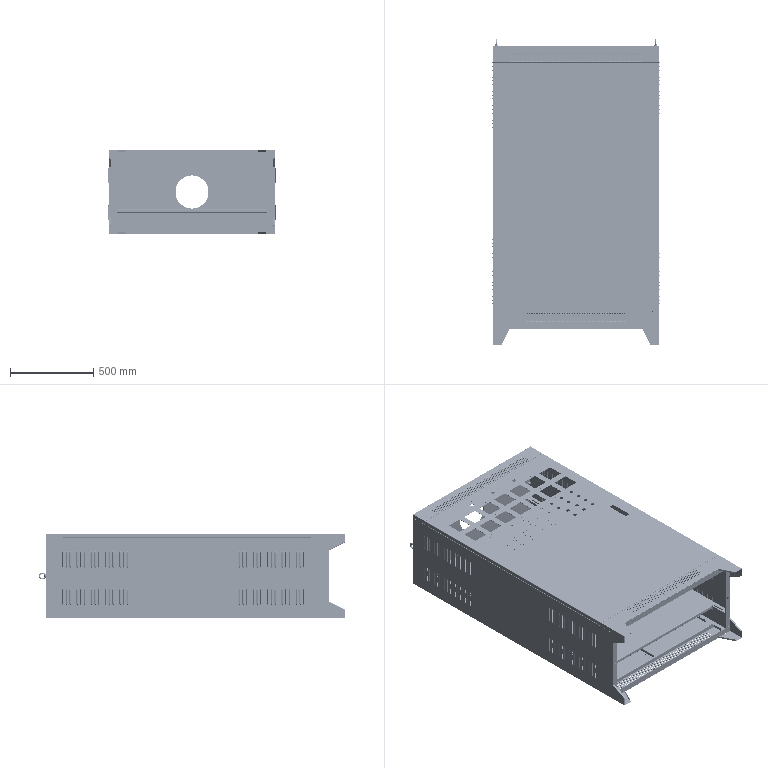Assembly | SolidWorks | mm | 36 component files | 42 solids | 7368 faces | box 1010 x 1843.66 x 510 mm | volume 13388712 mm3 | cylinder 3454 | plane 2960 | torus 460 | sphere 436 | spline 48 | cone 10 | commonest cylinder face diameters 6 x1184 8.4 x592 3.6 x592 3.4 x224 10 x216 8 x118 7.6 x108 12.4 x108
Bill of materials:
27x100IronPlate | 4 |  | Thin flat rectangular plate or strip, elongated, with no visible holes or cutouts.
AirFurnaceElectricalCabinet-AngleIronFrame | 2 |  | Rectangular open frame made of four straight bars of square-ish section, with one small round through-hole in each short side member.
AirFurnaceElectricalCabinet-DoorPanel | 1 |  | Flat rectangular plate with a cutout pattern in one region: two rows of seven square openings, a grid of small round holes below them, three larger round holes above, many tiny holes around the square openings, and one narrow rectangular slot.
AirFurnaceElectricalCabinet-WireDuct | 3 |  | Long, slender, shallow U-section (channel) profile of constant cross-section, with rounded inside corners.
AirFurnaceElectricalCabinet-WiringBoard | 2 |  | Thin sheet bent into a U shape: a flat base with two upright end flanges and small inside bend radii.
DoorPanelReinforcementPlate-L590 | 1 |  | Long hat-section (top-hat) rail: a recessed central channel with outward horizontal flanges on both sides and rounded bends.
DoorPanelReinforcementPlate-L790 | 1 |  | Long hat-section rail with a deep central channel, outward flanges and rounded bends; similar to the previous hat profile but longer relative to its section.
AirFurnaceElectricalCabinet-ElectricalPanel | 1 |  | Large flat rectangular sheet panel with shallow turned-down edges or lips, and small slots or notches spaced along the two long edges.
ElectricalPanelReinforcementPlate-L1425 | 2 |  | Long, narrow hat-section rail with outward flanges and rounded bends; a slimmer, longer version of the hat profile.
AirFurnaceElectricalCabinet-FrontDoorLowerPlate | 1 |  | Long, formed sheet strip with a stepped (Z-like) cross-section and a long row of narrow, closely spaced slots (louvre or vent pattern) in a slightly offset or embossed region.
AirFurnaceElectricalCabinet-LeftSidePlate | 1 |  | Rectangular sheet panel with short return flanges along the top and bottom long edges, and four groups of vertical louvre slots (two upper and two lower rows near each end), each group made of repeated sets of three slots.
AirFurnaceElectricalCabinet-RearLowerPlate | 1 |  | Long formed sheet strip with a flat base, a raised embossed area containing a long row of narrow transverse slots, and an upright side wall with a top flange turned outward at one edge.
AirFurnaceElectricalCabinet-RearSealingPlate | 1 |  | Thin flat rectangular plate with a small through hole near each of the four corners and a narrow stepped or lipped border around the edge.
DoorPanelReinforcementPlate-L1490 | 1 |  | Long, straight, constant-section profile with a hat (omega) cross-section: a raised flat top, two vertical walls, and a flat outward flange on each side, with rounded bends.
AirFurnaceElectricalCabinet-RightSidePlate | 1 |  | Long, sheet-metal-style panel with a C-like section. A flat web has short return flanges along the top and bottom edges, one with an extra small lip. Each end region has louver groups: two rows of four sets, each set made of three narrow vertical slots.
AirFurnaceElectricalCabinet-TopPlate | 1 |  | Channel-shaped sheet-metal bracket. A tall flat web has one large central round hole and a small round hole near each end. The top and bottom flanges have stepped returns, and each flange has a long row of small perforations.
BaseFoot-H100 | 4 |  | Bent sheet-metal piece with a tapered outline: a wide flange on top, a vertical web, and a short bottom flange. One edge is cut at an angle, so the plan outline is a trapezoid.
LargeLiftingRing | 2 |  | Eye-bolt-shaped part: a straight shank with external threads, a collar with a flared base, and a circular ring eye in a plane that contains the shank axis.
SealingPlateAngleIron | 4 |  | Flat right-triangle plate of uniform thickness with one round through hole near the corner where the two straight edges meet at a right angle.
UniversalAngleIron38x38x1690 | 2 |  | Long straight angle (L-section) with legs of about equal length, and a row of evenly spaced elongated slots along one leg.
Mates:
1. distance | AirFurnaceElectricalCabinet-LeftSidePlate-1 face at (-500, 1700, 229.2) dir (-1, 0, 0) | assembly plane at (0, 0, 0) dir (1, 0, 0)
2. coincident | AirFurnaceElectricalCabinet-AngleIronFrame-1 face at (-498.8, 0, 253.5) dir (0, -1, 0) | AirFurnaceElectricalCabinet-LeftSidePlate-1 face at (-498.05, 0, -253.6) dir (0, -1, 0)
3. distance | assembly plane at (0, 0, 0) dir (1, 0, 0) | AirFurnaceElectricalCabinet-RightSidePlate-1 face at (500, 1700, 229.2) dir (1, 0, 0)
4. coincident | AirFurnaceElectricalCabinet-AngleIronFrame-1 face at (495.5, 0, 253.5) dir (0, -1, 0) | AirFurnaceElectricalCabinet-RightSidePlate-1 face at (498.05, 0, 228) dir (0, -1, 0)
5. coincident | AirFurnaceElectricalCabinet-FrontDoorLowerPlate-1 plane at (0, 0, 255) dir (1, 0, 0) | assembly plane at (0, 0, 0) dir (1, 0, 0)
6. coincident | AirFurnaceElectricalCabinet-AngleIronFrame-1 face at (498.8, 0, 253.5) dir (0, -1, 0) | AirFurnaceElectricalCabinet-FrontDoorLowerPlate-1 plane at (0, 0, 255) dir (0, 1, 0)
7. distance | AirFurnaceElectricalCabinet-FrontDoorLowerPlate-1 face at (498.8, 0, 255) dir (0, 0, 1) | assembly plane at (0, 0, 0) dir (0, 0, 1)
8. coincident | AirFurnaceElectricalCabinet-RightSidePlate-1 face at (460, 1700, 229.2) dir (0, 0, 1) | AirFurnaceElectricalCabinet-FrontDoorLowerPlate-1 face at (498.8, 100, 229.2) dir (0, 0, 1)
9. coincident | AirFurnaceElectricalCabinet-LeftSidePlate-1 face at (-460, 1700, 229.2) dir (0, 0, 1) | AirFurnaceElectricalCabinet-FrontDoorLowerPlate-1 face at (498.8, 100, 229.2) dir (0, 0, 1)
10. coincident | AirFurnaceElectricalCabinet-TopPlate-2 plane at (0, 1700, 0) dir (1, 0, 0) | assembly plane at (0, 0, 0) dir (1, 0, 0)
11. coincident | AirFurnaceElectricalCabinet-FrontDoorLowerPlate-1 face at (498.8, 0, 255) dir (0, 0, 1) | AirFurnaceElectricalCabinet-TopPlate-2 face at (498.8, 1600, 255) dir (0, 0, 1)
12. distance | AirFurnaceElectricalCabinet-AngleIronFrame-1 face at (498.8, 0, 253.5) dir (0, -1, 0) | AirFurnaceElectricalCabinet-TopPlate-2 face at (498.8, 1700, 255) dir (0, 1, 0)
13. coincident | AirFurnaceElectricalCabinet-RearLowerPlate-1 plane at (0, 0, -255) dir (1, 0, 0) | assembly plane at (0, 0, 0) dir (1, 0, 0)
14. coincident | AirFurnaceElectricalCabinet-AngleIronFrame-1 face at (495.5, 0, -253.5) dir (0, -1, 0) | AirFurnaceElectricalCabinet-RearLowerPlate-1 plane at (0, 0, -255) dir (0, 1, 0)
15. coincident | AirFurnaceElectricalCabinet-TopPlate-2 face at (498.8, 1700, -255) dir (0, 0, -1) | AirFurnaceElectricalCabinet-RearLowerPlate-1 face at (460, 0, -255) dir (0, 0, -1)
16. coincident | AirFurnaceElectricalCabinet-TopPlate-2 face at (498.8, 1698.8, 255) dir (0, -1, 0) | AirFurnaceElectricalCabinet-AngleIronFrame-2 face at (-495.5, 1698.8, -253.8) dir (0, 1, 0)
17. coincident | AirFurnaceElectricalCabinet-AngleIronFrame-2 plane at (0, 1698.8, -0.3) dir (-1, 0, 0) | assembly plane at (0, 0, 0) dir (1, 0, 0)
18. coincident | AirFurnaceElectricalCabinet-TopPlate-2 face at (498.8, 1700, -253.8) dir (0, 0, 1) | AirFurnaceElectricalCabinet-AngleIronFrame-2 face at (-495.5, 1660.8, -253.8) dir (0, 0, -1)
19. coincident | AirFurnaceElectricalCabinet-AngleIronFrame-1 face at (498.8, 3, 253.5) dir (0, 1, 0) | UniversalAngleIron38x38x1690-1 face at (457.8, 3, -108) dir (0, -1, 0)
20. distance | UniversalAngleIron38x38x1690-1 face at (495.8, 1693, -105) dir (0, 0, 1) | AirFurnaceElectricalCabinet-TopPlate-2 face at (498.8, 1700, -255) dir (0, 0, -1)
21. coincident | AirFurnaceElectricalCabinet-ElectricalPanelAssembly-1 plane at (0, 835.8, -103.5) dir (1, 0, 0) | assembly plane at (0, 0, 0) dir (1, 0, 0)
22. coincident | UniversalAngleIron38x38x1690-2 face at (-495.8, 3, -105) dir (0, 0, 1) | AirFurnaceElectricalCabinet-ElectricalPanelAssembly-1/AirFurnaceElectricalCabinet-ElectricalPanel-1 face at (487.5, 1560.8, -105) dir (0, 0, -1)
23. coincident | AirFurnaceElectricalCabinet-RearLowerPlate-1 face at (460, 110.8, -228) dir (0, 1, 0) | AirFurnaceElectricalCabinet-ElectricalPanelAssembly-1/AirFurnaceElectricalCabinet-ElectricalPanel-1 face at (487.5, 110.8, -103.5) dir (0, -1, 0)
24. coincident | AirFurnaceElectricalCabinet-FrontDoorLowerPlate-1 face at (498.8, 0, 255) dir (0, 0, 1) | BaseFoot-H100-1 face at (-500, -100, 255) dir (0, 0, 1)
25. coincident | AirFurnaceElectricalCabinet-LeftSidePlate-1 face at (-500, 1700, 229.2) dir (-1, 0, 0) | BaseFoot-H100-1 face at (-500, -100, 155) dir (-1, 0, 0)
26. coincident | AirFurnaceElectricalCabinet-RightSidePlate-1 face at (500, 1700, 229.2) dir (1, 0, 0) | BaseFoot-H100-2 face at (500, -100, 255) dir (1, 0, 0)
27. coincident | AirFurnaceElectricalCabinet-FrontDoorLowerPlate-1 face at (498.8, 0, 255) dir (0, 0, 1) | BaseFoot-H100-2 face at (400, -100, 255) dir (0, 0, 1)
28. coincident | AirFurnaceElectricalCabinet-AngleIronFrame-1 face at (498.8, 0, 253.5) dir (0, -1, 0) | BaseFoot-H100-2 edge at (498.8, 0, 252.8) dir (0, 0, -1)
29. coincident | AirFurnaceElectricalCabinet-AngleIronFrame-1 face at (495.5, 0, 253.5) dir (0, -1, 0) | BaseFoot-H100-1 face at (-497.8, 0, 252.8) dir (0, 1, 0)
30. coincident | AirFurnaceElectricalCabinet-RightSidePlate-1 face at (500, 1700, 229.2) dir (1, 0, 0) | BaseFoot-H100-3 face at (500, -100, -155) dir (1, 0, 0)
31. coincident | AirFurnaceElectricalCabinet-RearLowerPlate-1 face at (460, 0, -255) dir (0, 0, -1) | BaseFoot-H100-3 face at (500, -100, -255) dir (0, 0, -1)
32. coincident | AirFurnaceElectricalCabinet-AngleIronFrame-1 face at (495.5, 0, -253.5) dir (0, -1, 0) | BaseFoot-H100-3 face at (497.8, 0, -252.8) dir (0, 1, 0)
33. coincident | AirFurnaceElectricalCabinet-LeftSidePlate-1 face at (-500, 1700, 229.2) dir (-1, 0, 0) | BaseFoot-H100-4 face at (-500, -100, -255) dir (-1, 0, 0)
34. coincident | AirFurnaceElectricalCabinet-RearLowerPlate-1 face at (460, 0, -255) dir (0, 0, -1) | BaseFoot-H100-4 face at (-400, -100, -255) dir (0, 0, -1)
35. coincident | AirFurnaceElectricalCabinet-AngleIronFrame-1 face at (495.5, 0, -253.5) dir (0, -1, 0) | BaseFoot-H100-4 edge at (-400, 0, -255) dir (-1, 0, 0)
36. coincident | AirFurnaceElectricalCabinet-TopPlate-2 face at (498.8, 1600, 255) dir (0, 0, 1) | AirFurnaceElectricalCabinet-DoorPanelAssembly-1/AirFurnaceElectricalCabinet-DoorPanel-1 face at (0, 850, 255) dir (0, 0, 1)
37. distance | AirFurnaceElectricalCabinet-FrontDoorLowerPlate-1 face at (498.8, 100, 255) dir (0, 1, 0) | AirFurnaceElectricalCabinet-DoorPanelAssembly-1/AirFurnaceElectricalCabinet-DoorPanel-1 face at (0, 102, 255) dir (0, -1, 0)
38. concentric | AirFurnaceElectricalCabinet-FrontDoorLowerPlate-1 face at (-493, 98.8, 248) dir (0, 1, 0) r 3.25 | AirFurnaceElectricalCabinet-DoorPanelAssembly-1/AirFurnaceElectricalCabinet-DoorPanel-1 face at (-493, 101.996, 248) dir (0, 1, 0) r 3.25
39. coincident | AirFurnaceElectricalCabinet-LeftSidePlate-1 face at (-460, 1700, -227.8) dir (0, 0, 1) | SealingPlateAngleIron-1 face at (-460, 100, -227.8) dir (0, 0, -1)
40. coincident | AirFurnaceElectricalCabinet-LeftSidePlate-1 face at (-460, 1700, -254.8) dir (1, 0, 0) | SealingPlateAngleIron-1 face at (-460, 165, -227.8) dir (-1, 0, 0)
41. coincident | AirFurnaceElectricalCabinet-RearLowerPlate-1 face at (460, 100, -255) dir (0, 1, 0) | SealingPlateAngleIron-1 face at (-460, 100, -227.8) dir (0, -1, 0)
42. coincident | SealingPlateAngleIron-1 face at (-460, 100, -227.8) dir (0, 0, -1) | SealingPlateAngleIron-2 face at (-460, 1600, -227.8) dir (0, 0, -1)
43. coincident | AirFurnaceElectricalCabinet-TopPlate-2 face at (498.8, 1600, -255) dir (0, -1, 0) | SealingPlateAngleIron-2 face at (-395, 1600, -227.8) dir (0, 1, 0)
44. coincident | AirFurnaceElectricalCabinet-LeftSidePlate-1 face at (-460, 1700, -254.8) dir (1, 0, 0) | SealingPlateAngleIron-2 face at (-460, 1600, -227.8) dir (-1, 0, 0)
45. coincident | AirFurnaceElectricalCabinet-RearSealingPlateAssembly-1 plane at (0, 850, -255) dir (-1, 0, 0) | assembly plane at (0, 0, 0) dir (1, 0, 0)
46. coincident | AirFurnaceElectricalCabinet-TopPlate-2 face at (498.8, 1700, -255) dir (0, 0, -1) | AirFurnaceElectricalCabinet-RearSealingPlateAssembly-1/AirFurnaceElectricalCabinet-RearSealingPlate-1 face at (0, 850, -255) dir (0, 0, -1)
47. distance | AirFurnaceElectricalCabinet-TopPlate-2 face at (498.8, 1600, -255) dir (0, -1, 0) | AirFurnaceElectricalCabinet-RearSealingPlateAssembly-1/AirFurnaceElectricalCabinet-RearSealingPlate-1 face at (0, 1598.5, -255) dir (0, 1, 0)
48. coincident | AirFurnaceElectricalCabinet-RightSidePlate-1 face at (500, 1700, 229.2) dir (1, 0, 0) | 27x100IronPlate-1 face at (500, 50, 242.1) dir (1, 0, 0)
49. coincident | AirFurnaceElectricalCabinet-FrontDoorLowerPlate-1 face at (498.8, 100, 255) dir (0, 1, 0) | 27x100IronPlate-1 face at (498.8, 100, 255) dir (0, 1, 0)
50. coincident | AirFurnaceElectricalCabinet-FrontDoorLowerPlate-1 face at (498.8, 0, 255) dir (0, 0, 1) | 27x100IronPlate-1 face at (498.8, 100, 255) dir (0, 0, 1)
51. coincident | AirFurnaceElectricalCabinet-RightSidePlate-1 face at (500, 1700, 229.2) dir (1, 0, 0) | 27x100IronPlate-2 face at (500, 1650, 242.1) dir (1, 0, 0)
52. coincident | AirFurnaceElectricalCabinet-FrontDoorLowerPlate-1 face at (498.8, 0, 255) dir (0, 0, 1) | 27x100IronPlate-2 face at (498.8, 1700, 255) dir (0, 0, 1)
53. coincident | AirFurnaceElectricalCabinet-TopPlate-2 face at (498.8, 1700, 255) dir (0, 1, 0) | 27x100IronPlate-2 face at (498.8, 1700, 255) dir (0, 1, 0)
54. coincident | AirFurnaceElectricalCabinet-AngleIronFrame-1 face at (495.8, 38, 253.5) dir (-1, 0, 0) | UniversalAngleIron38x38x1690-1 face at (495.8, 1693, -143) dir (1, 0, 0)
55. concentric | AirFurnaceElectricalCabinet-TopPlate-2 face at (-479.8, 1698.8, 0) dir (0, 1, 0) r 7.75 | LargeLiftingRing-1 face at (-479.8, 1680, 0) dir (0, 1, 0) r 7
56. coincident | AirFurnaceElectricalCabinet-TopPlate-2 face at (498.8, 1700, 255) dir (0, 1, 0) | LargeLiftingRing-1 face at (-479.8, 1700, 0) dir (0, -1, 0)
57. parallel | LargeLiftingRing-1 plane at (-479.8, 1722.5, 0) dir (1, 0, 0) | assembly plane at (0, 0, 0) dir (1, 0, 0)
58. coincident | AirFurnaceElectricalCabinet-DoorPanel-1 face at (0, 0, -1.5) dir (0, 0, -1) | DoorPanelReinforcementPlate-L790-1 face at (-495, -116.5, -1.5) dir (0, 0, 1)
59. coincident | AirFurnaceElectricalCabinet-DoorPanel-1 face at (0, 0, -1.5) dir (0, 0, -1) | DoorPanelReinforcementPlate-L590-1 face at (-30.8, -156.5, -1.5) dir (0, 0, 1)
60. coincident | DoorPanelReinforcementPlate-L790-1 plane at (0, -136.5, -2.7) dir (-1, 0, 0) | AirFurnaceElectricalCabinet-DoorPanelAssembly plane at (0, 0, 0) dir (1, 0, 0)
61. coincident | DoorPanelReinforcementPlate-L590-1 plane at (0, -451.5, -2.7) dir (-1, 0, 0) | AirFurnaceElectricalCabinet-DoorPanelAssembly plane at (0, 0, 0) dir (1, 0, 0)
62. coincident | AirFurnaceElectricalCabinet-DoorPanel-1 face at (0, -746.5, 0) dir (0, 1, 0) | DoorPanelReinforcementPlate-L590-1 face at (20.75, -746.5, -1.5) dir (0, -1, 0)
63. coincident | DoorPanelReinforcementPlate-L790-1 face at (-495, -156.5, -2.7) dir (0, -1, 0) | DoorPanelReinforcementPlate-L590-1 face at (18.05, -156.5, -18.3) dir (0, 1, 0)
64. coincident | AirFurnaceElectricalCabinet-DoorPanel-1 face at (0, 0, -1.5) dir (0, 0, -1) | AirFurnaceElectricalCabinet-WireDuct-1 face at (-400, 511, -1.5) dir (0, 0, 1)
65. coincident | AirFurnaceElectricalCabinet-WireDuct-1 plane at (0, 501, -9.5) dir (-1, 0, 0) | AirFurnaceElectricalCabinet-DoorPanelAssembly plane at (0, 0, 0) dir (1, 0, 0)
66. distance | AirFurnaceElectricalCabinet-WireDuct-1 plane at (0, 501, -9.5) dir (0, 1, 0) | AirFurnaceElectricalCabinet-DoorPanel-1 face at (209.86, 481, -1.5) dir (0, -1, 0)
67. coincident | AirFurnaceElectricalCabinet-DoorPanel-1 face at (0, 0, -1.5) dir (0, 0, -1) | AirFurnaceElectricalCabinet-WireDuct-2 face at (-400, 319, -1.5) dir (0, 0, 1)
68. coincident | AirFurnaceElectricalCabinet-WireDuct-2 plane at (0, 309, -9.5) dir (-1, 0, 0) | AirFurnaceElectricalCabinet-DoorPanelAssembly plane at (0, 0, 0) dir (1, 0, 0)
69. coincident | AirFurnaceElectricalCabinet-DoorPanel-1 face at (0, 0, -1.5) dir (0, 0, -1) | AirFurnaceElectricalCabinet-WireDuct-3 face at (-400, 139, -1.5) dir (0, 0, 1)
70. coincident | AirFurnaceElectricalCabinet-WireDuct-3 plane at (0, 129, -9.5) dir (-1, 0, 0) | AirFurnaceElectricalCabinet-DoorPanelAssembly plane at (0, 0, 0) dir (1, 0, 0)
71. coincident | AirFurnaceElectricalCabinet-DoorPanel-1 face at (0, 0, -1.5) dir (0, 0, -1) | AirFurnaceElectricalCabinet-WiringBoard-1 face at (-470, 551, -1.5) dir (0, 0, 1)
72. distance | AirFurnaceElectricalCabinet-WiringBoard-1 plane at (-460, 501, -25) dir (-1, 0, 0) | AirFurnaceElectricalCabinet-DoorPanelAssembly plane at (0, 0, 0) dir (1, 0, 0)
73. coincident | AirFurnaceElectricalCabinet-WireDuct-1 plane at (0, 501, -9.5) dir (0, 1, 0) | AirFurnaceElectricalCabinet-WiringBoard-1 plane at (-460, 501, -25) dir (0, 1, 0)
74. coincident | AirFurnaceElectricalCabinet-WiringBoard-1 plane at (-460, 501, -25) dir (-1, 0, 0) | AirFurnaceElectricalCabinet-WiringBoard-2 plane at (-460, 309, -25) dir (-1, 0, 0)
75. coincident | AirFurnaceElectricalCabinet-WiringBoard-1 face at (-470, 451, -25) dir (0, 0, -1) | AirFurnaceElectricalCabinet-WiringBoard-2 face at (-470, 259, -25) dir (0, 0, -1)
76. coincident | AirFurnaceElectricalCabinet-WireDuct-2 plane at (0, 309, -9.5) dir (0, 1, 0) | AirFurnaceElectricalCabinet-WiringBoard-2 plane at (-460, 309, -25) dir (0, 1, 0)
77. distance | AirFurnaceElectricalCabinet-DoorPanel-1 face at (209.86, 389, -1.5) dir (0, 1, 0) | AirFurnaceElectricalCabinet-WireDuct-2 plane at (0, 309, -9.5) dir (0, 1, 0)
78. distance | AirFurnaceElectricalCabinet-WireDuct-2 plane at (0, 309, -9.5) dir (0, 1, 0) | AirFurnaceElectricalCabinet-WireDuct-3 plane at (0, 129, -9.5) dir (0, 1, 0)
79. coincident | AirFurnaceElectricalCabinet-ElectricalPanel-1 face at (487.5, 725, -1.5) dir (0, 0, -1) | ElectricalPanelReinforcementPlate-L1425-1 face at (175, -712.5, -1.5) dir (0, 0, 1)
80. coincident | ElectricalPanelReinforcementPlate-L1425-1 plane at (200, 0, -2.7) dir (0, -1, 0) | AirFurnaceElectricalCabinet-ElectricalPanelAssembly plane at (0, 0, 0) dir (0, 1, 0)
81. distance | ElectricalPanelReinforcementPlate-L1425-1 plane at (200, 0, -2.7) dir (1, 0, 0) | AirFurnaceElectricalCabinet-ElectricalPanelAssembly plane at (0, 0, 0) dir (1, 0, 0)
82. coincident | DoorPanelReinforcementPlate-L1490-1 plane at (0, 0, -2.7) dir (-1, 0, 0) | AirFurnaceElectricalCabinet-RearSealingPlateAssembly plane at (0, 0, 0) dir (1, 0, 0)
83. coincident | AirFurnaceElectricalCabinet-RearSealingPlate-1 face at (0, 0, -1.5) dir (0, 0, -1) | DoorPanelReinforcementPlate-L1490-1 face at (25, 745, -1.5) dir (0, 0, 1)
84. coincident | DoorPanelReinforcementPlate-L1490-1 plane at (0, 0, -2.7) dir (0, 1, 0) | AirFurnaceElectricalCabinet-RearSealingPlateAssembly plane at (0, 0, 0) dir (0, 1, 0)